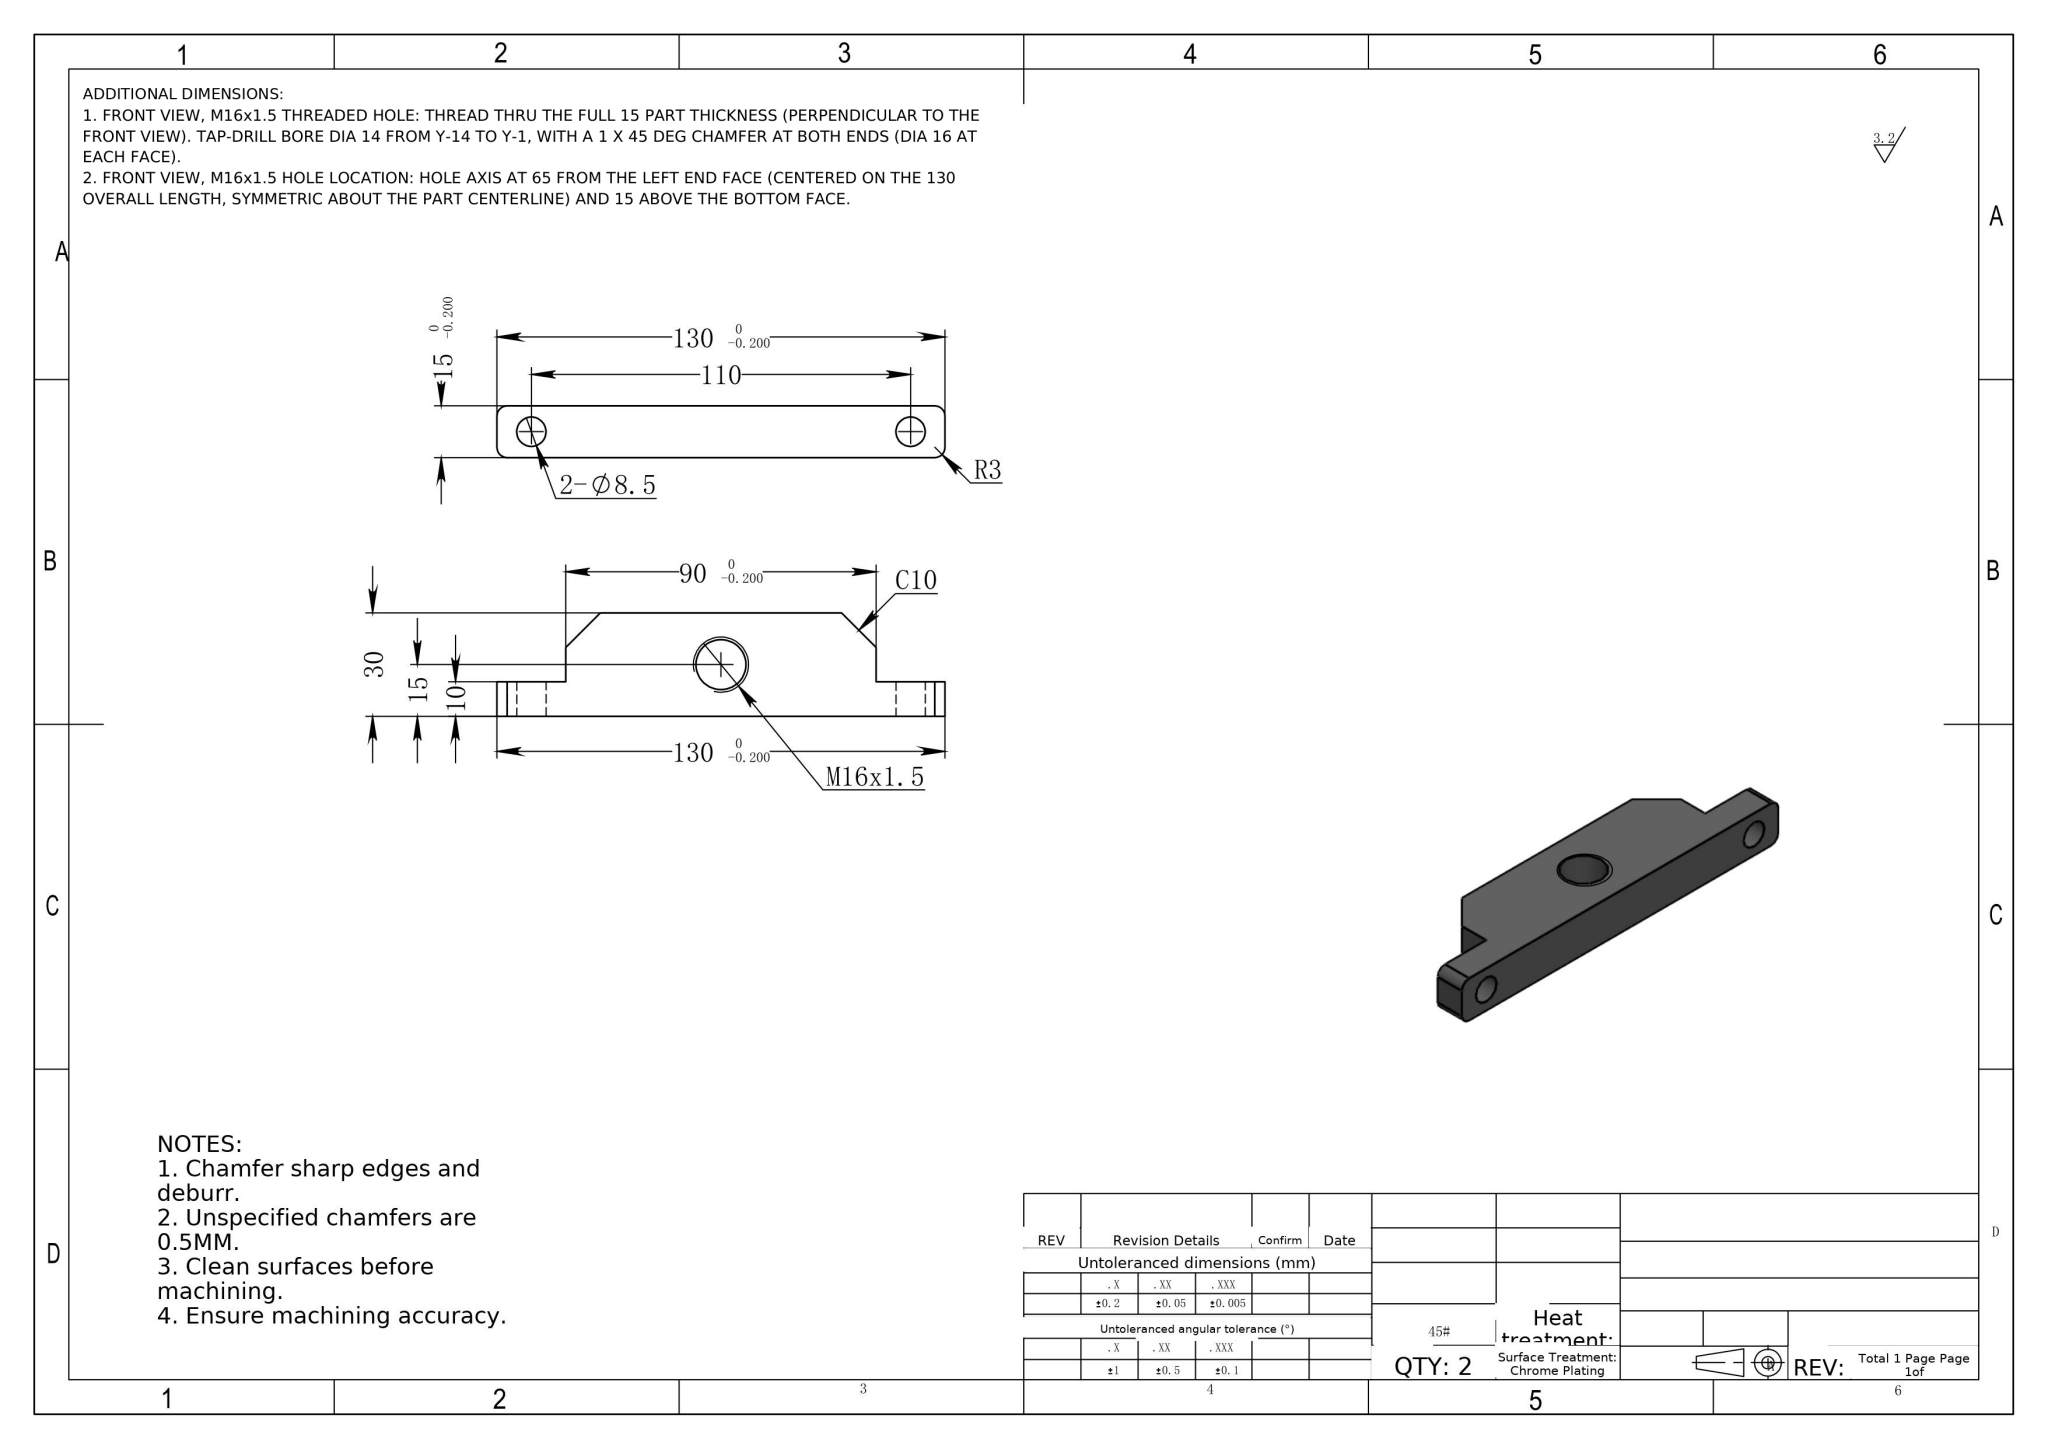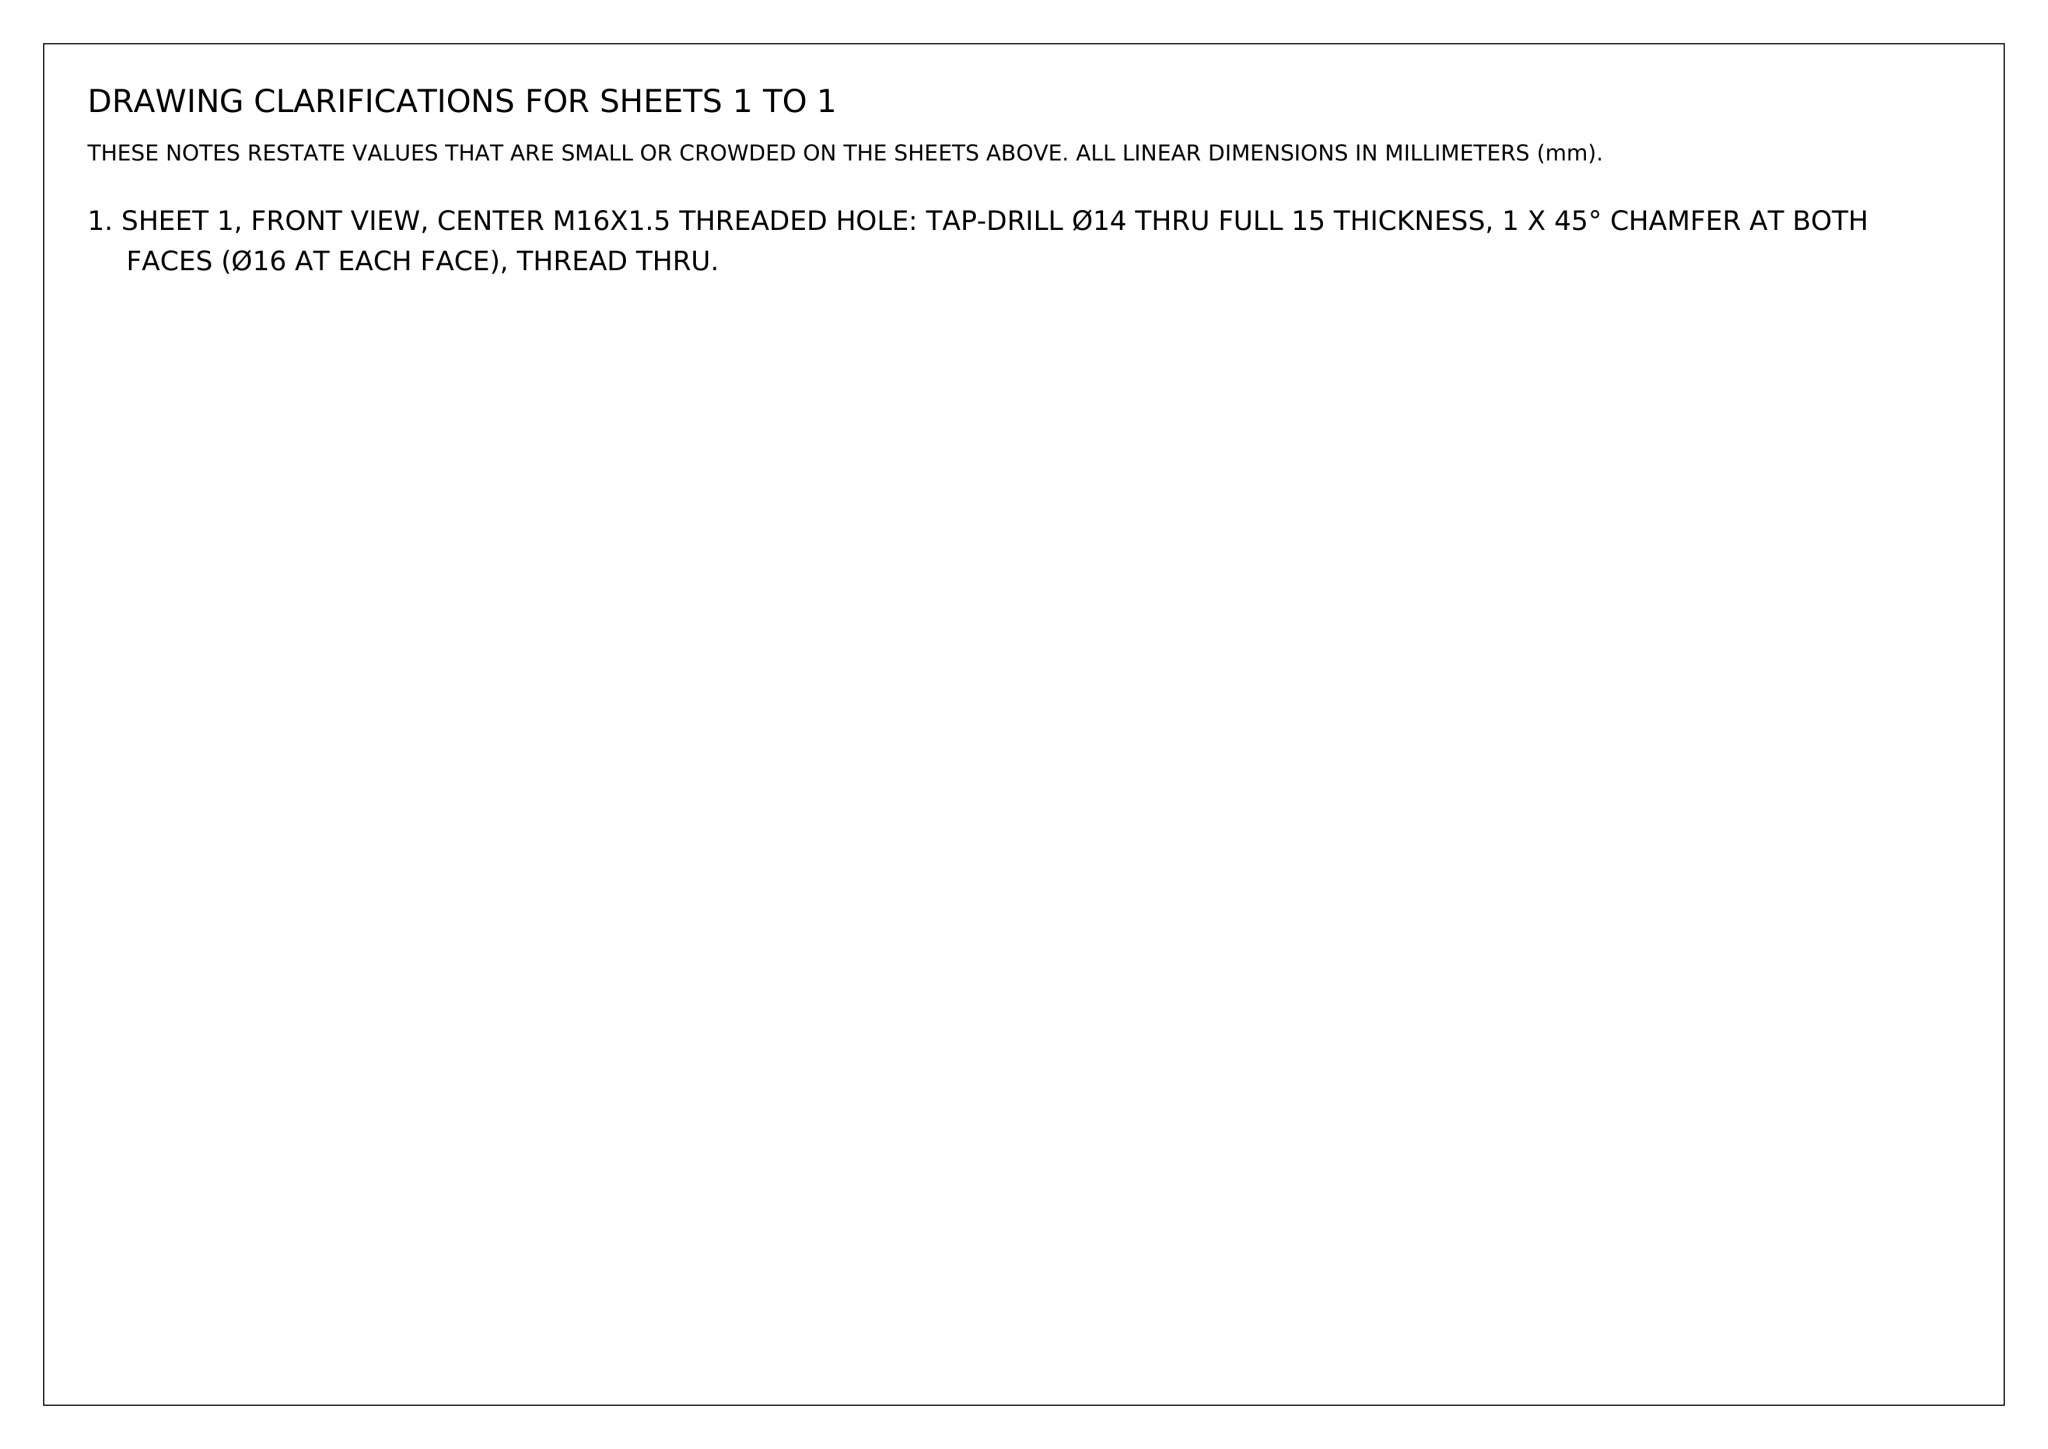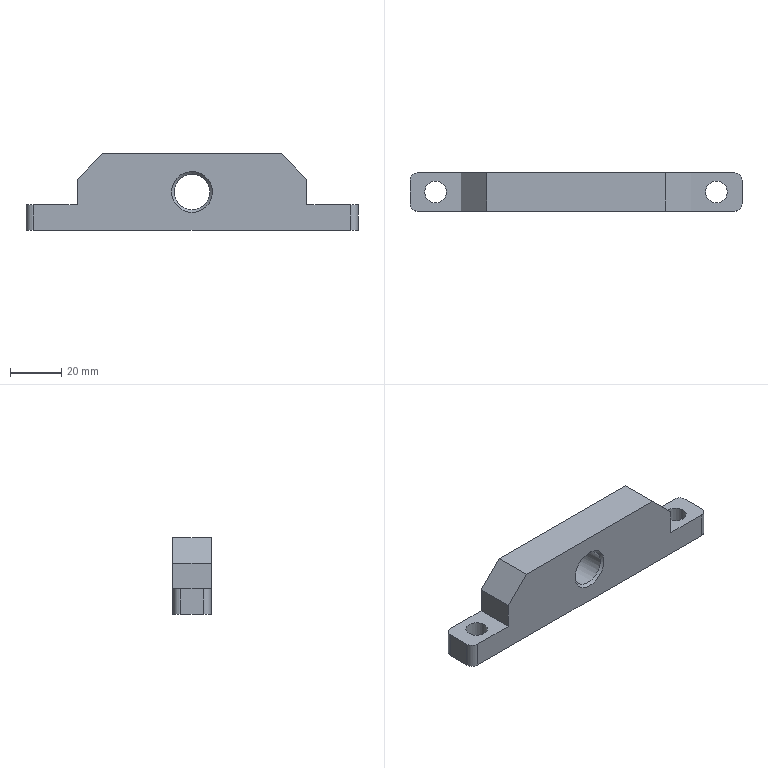Part | NX | mm | Offset Dual-Ear Mounting Bar | 1 solid | 21 faces | box 130 x 15 x 30 mm | volume 41433 mm3 | plane 12 | cylinder 7 | cone 2 | commonest cylinder face diameters 6 x4 8.5 x2 14 x1
STEP:
#1=CARTESIAN_POINT('',(0.,0.,0.));
#2=DIRECTION('',(0.,0.,1.));
#3=DIRECTION('',(1.,0.,0.));
#4=AXIS2_PLACEMENT_3D('',#1,#2,#3);
#5=(LENGTH_UNIT()NAMED_UNIT(*)SI_UNIT(.MILLI.,.METRE.));
#6=UNCERTAINTY_MEASURE_WITH_UNIT(LENGTH_MEASURE(0.00002),#5,'','');
#7=(NAMED_UNIT(*)PLANE_ANGLE_UNIT()SI_UNIT($,.RADIAN.));
#8=PLANE_ANGLE_MEASURE_WITH_UNIT(PLANE_ANGLE_MEASURE(0.01745),#7);
#9=DIMENSIONAL_EXPONENTS(0.,0.,0.,0.,0.,0.,0.);
#10=(CONVERSION_BASED_UNIT('',#8)NAMED_UNIT(#9)PLANE_ANGLE_UNIT());
#11=(NAMED_UNIT(*)SI_UNIT($,.STERADIAN.)SOLID_ANGLE_UNIT());
#12=(GEOMETRIC_REPRESENTATION_CONTEXT(3)GLOBAL_UNCERTAINTY_ASSIGNED_CONTEXT((#6))GLOBAL_UNIT_ASSIGNED_CONTEXT((#5,#10,#11))REPRESENTATION_CONTEXT('',''));
#13=SHAPE_REPRESENTATION('',(#4),#12);
#14=CARTESIAN_POINT('',(14.25,-7.5,10.));
#15=VERTEX_POINT('',#14);
#16=CARTESIAN_POINT('',(10.,-7.5,10.));
#17=DIRECTION('',(0.,0.,1.));
#18=DIRECTION('',(1.,0.,0.));
#19=AXIS2_PLACEMENT_3D('',#16,#17,#18);
#20=CIRCLE('',#19,4.25);
#21=EDGE_CURVE('',#15,#15,#20,.T.);
#22=ORIENTED_EDGE('',*,*,#21,.F.);
#23=EDGE_LOOP('',(#22));
#24=FACE_BOUND('',#23,.T.);
#25=CARTESIAN_POINT('',(20.,0.,10.));
#26=VERTEX_POINT('',#25);
#27=CARTESIAN_POINT('',(20.,-15.,10.));
#28=VERTEX_POINT('',#27);
#29=CARTESIAN_POINT('',(20.,0.,10.));
#30=DIRECTION('',(0.,-1.,0.));
#31=VECTOR('',#30,1.);
#32=LINE('',#29,#31);
#33=EDGE_CURVE('',#26,#28,#32,.T.);
#34=ORIENTED_EDGE('',*,*,#33,.F.);
#35=CARTESIAN_POINT('',(3.,0.,10.));
#36=VERTEX_POINT('',#35);
#37=CARTESIAN_POINT('',(130.,0.,10.));
#38=DIRECTION('',(-1.,-0.,0.));
#39=VECTOR('',#38,1.);
#40=LINE('',#37,#39);
#41=EDGE_CURVE('',#26,#36,#40,.T.);
#42=ORIENTED_EDGE('',*,*,#41,.T.);
#43=CARTESIAN_POINT('',(0.,-3.,10.));
#44=VERTEX_POINT('',#43);
#45=CARTESIAN_POINT('',(3.,-3.,10.));
#46=DIRECTION('',(0.,0.,1.));
#47=DIRECTION('',(1.,0.,0.));
#48=AXIS2_PLACEMENT_3D('',#45,#46,#47);
#49=CIRCLE('',#48,3.);
#50=EDGE_CURVE('',#36,#44,#49,.T.);
#51=ORIENTED_EDGE('',*,*,#50,.T.);
#52=CARTESIAN_POINT('',(0.,-12.,10.));
#53=VERTEX_POINT('',#52);
#54=CARTESIAN_POINT('',(0.,0.,10.));
#55=DIRECTION('',(0.,-1.,0.));
#56=VECTOR('',#55,1.);
#57=LINE('',#54,#56);
#58=EDGE_CURVE('',#44,#53,#57,.T.);
#59=ORIENTED_EDGE('',*,*,#58,.T.);
#60=CARTESIAN_POINT('',(3.,-15.,10.));
#61=VERTEX_POINT('',#60);
#62=CARTESIAN_POINT('',(3.,-12.,10.));
#63=DIRECTION('',(0.,0.,1.));
#64=DIRECTION('',(1.,0.,0.));
#65=AXIS2_PLACEMENT_3D('',#62,#63,#64);
#66=CIRCLE('',#65,3.);
#67=EDGE_CURVE('',#53,#61,#66,.T.);
#68=ORIENTED_EDGE('',*,*,#67,.T.);
#69=CARTESIAN_POINT('',(0.,-15.,10.));
#70=DIRECTION('',(1.,0.,0.));
#71=VECTOR('',#70,1.);
#72=LINE('',#69,#71);
#73=EDGE_CURVE('',#61,#28,#72,.T.);
#74=ORIENTED_EDGE('',*,*,#73,.T.);
#75=EDGE_LOOP('',(#34,#42,#51,#59,#68,#74));
#76=FACE_BOUND('',#75,.T.);
#77=CARTESIAN_POINT('',(0.,0.,10.));
#78=DIRECTION('',(0.,0.,1.));
#79=DIRECTION('',(1.,0.,0.));
#80=AXIS2_PLACEMENT_3D('',#77,#78,#79);
#81=PLANE('',#80);
#82=ADVANCED_FACE('',(#24,#76),#81,.T.);
#83=ORIENTED_EDGE('',*,*,#58,.F.);
#84=CARTESIAN_POINT('',(0.,-3.,0.));
#85=VERTEX_POINT('',#84);
#86=CARTESIAN_POINT('',(0.,-3.,10.));
#87=DIRECTION('',(0.,0.,-1.));
#88=VECTOR('',#87,1.);
#89=LINE('',#86,#88);
#90=EDGE_CURVE('',#44,#85,#89,.T.);
#91=ORIENTED_EDGE('',*,*,#90,.T.);
#92=CARTESIAN_POINT('',(0.,-12.,0.));
#93=VERTEX_POINT('',#92);
#94=CARTESIAN_POINT('',(0.,0.,0.));
#95=DIRECTION('',(0.,-1.,0.));
#96=VECTOR('',#95,1.);
#97=LINE('',#94,#96);
#98=EDGE_CURVE('',#85,#93,#97,.T.);
#99=ORIENTED_EDGE('',*,*,#98,.T.);
#100=CARTESIAN_POINT('',(0.,-12.,10.));
#101=DIRECTION('',(0.,0.,1.));
#102=VECTOR('',#101,1.);
#103=LINE('',#100,#102);
#104=EDGE_CURVE('',#93,#53,#103,.T.);
#105=ORIENTED_EDGE('',*,*,#104,.T.);
#106=EDGE_LOOP('',(#83,#91,#99,#105));
#107=FACE_OUTER_BOUND('',#106,.T.);
#108=CARTESIAN_POINT('',(0.,0.,10.));
#109=DIRECTION('',(1.,0.,0.));
#110=DIRECTION('',(0.,0.,-1.));
#111=AXIS2_PLACEMENT_3D('',#108,#109,#110);
#112=PLANE('',#111);
#113=ADVANCED_FACE('',(#107),#112,.F.);
#114=CARTESIAN_POINT('',(57.,-15.,15.));
#115=VERTEX_POINT('',#114);
#116=CARTESIAN_POINT('',(65.,-15.,15.));
#117=DIRECTION('',(-0.,1.,0.));
#118=DIRECTION('',(-1.,-0.,0.));
#119=AXIS2_PLACEMENT_3D('',#116,#117,#118);
#120=CIRCLE('',#119,8.);
#121=EDGE_CURVE('',#115,#115,#120,.T.);
#122=ORIENTED_EDGE('',*,*,#121,.T.);
#123=EDGE_LOOP('',(#122));
#124=FACE_BOUND('',#123,.T.);
#125=CARTESIAN_POINT('',(110.,-15.,20.));
#126=VERTEX_POINT('',#125);
#127=CARTESIAN_POINT('',(110.,-15.,10.));
#128=VERTEX_POINT('',#127);
#129=CARTESIAN_POINT('',(110.,-15.,30.));
#130=DIRECTION('',(0.,0.,-1.));
#131=VECTOR('',#130,1.);
#132=LINE('',#129,#131);
#133=EDGE_CURVE('',#126,#128,#132,.T.);
#134=ORIENTED_EDGE('',*,*,#133,.F.);
#135=CARTESIAN_POINT('',(100.,-15.,30.));
#136=VERTEX_POINT('',#135);
#137=CARTESIAN_POINT('',(100.,-15.,30.));
#138=DIRECTION('',(-0.7071,-0.,0.7071));
#139=VECTOR('',#138,1.);
#140=LINE('',#137,#139);
#141=EDGE_CURVE('',#126,#136,#140,.T.);
#142=ORIENTED_EDGE('',*,*,#141,.T.);
#143=CARTESIAN_POINT('',(30.,-15.,30.));
#144=VERTEX_POINT('',#143);
#145=CARTESIAN_POINT('',(20.,-15.,30.));
#146=DIRECTION('',(1.,0.,0.));
#147=VECTOR('',#146,1.);
#148=LINE('',#145,#147);
#149=EDGE_CURVE('',#144,#136,#148,.T.);
#150=ORIENTED_EDGE('',*,*,#149,.F.);
#151=CARTESIAN_POINT('',(20.,-15.,20.));
#152=VERTEX_POINT('',#151);
#153=CARTESIAN_POINT('',(30.,-15.,30.));
#154=DIRECTION('',(-0.7071,-0.,-0.7071));
#155=VECTOR('',#154,1.);
#156=LINE('',#153,#155);
#157=EDGE_CURVE('',#144,#152,#156,.T.);
#158=ORIENTED_EDGE('',*,*,#157,.T.);
#159=CARTESIAN_POINT('',(20.,-15.,30.));
#160=DIRECTION('',(0.,0.,-1.));
#161=VECTOR('',#160,1.);
#162=LINE('',#159,#161);
#163=EDGE_CURVE('',#152,#28,#162,.T.);
#164=ORIENTED_EDGE('',*,*,#163,.T.);
#165=ORIENTED_EDGE('',*,*,#73,.F.);
#166=CARTESIAN_POINT('',(3.,-15.,0.));
#167=VERTEX_POINT('',#166);
#168=CARTESIAN_POINT('',(3.,-15.,10.));
#169=DIRECTION('',(0.,0.,-1.));
#170=VECTOR('',#169,1.);
#171=LINE('',#168,#170);
#172=EDGE_CURVE('',#61,#167,#171,.T.);
#173=ORIENTED_EDGE('',*,*,#172,.T.);
#174=CARTESIAN_POINT('',(127.,-15.,0.));
#175=VERTEX_POINT('',#174);
#176=CARTESIAN_POINT('',(0.,-15.,0.));
#177=DIRECTION('',(1.,0.,0.));
#178=VECTOR('',#177,1.);
#179=LINE('',#176,#178);
#180=EDGE_CURVE('',#167,#175,#179,.T.);
#181=ORIENTED_EDGE('',*,*,#180,.T.);
#182=CARTESIAN_POINT('',(127.,-15.,10.));
#183=VERTEX_POINT('',#182);
#184=CARTESIAN_POINT('',(127.,-15.,10.));
#185=DIRECTION('',(0.,0.,1.));
#186=VECTOR('',#185,1.);
#187=LINE('',#184,#186);
#188=EDGE_CURVE('',#175,#183,#187,.T.);
#189=ORIENTED_EDGE('',*,*,#188,.T.);
#190=CARTESIAN_POINT('',(0.,-15.,10.));
#191=DIRECTION('',(1.,0.,0.));
#192=VECTOR('',#191,1.);
#193=LINE('',#190,#192);
#194=EDGE_CURVE('',#128,#183,#193,.T.);
#195=ORIENTED_EDGE('',*,*,#194,.F.);
#196=EDGE_LOOP('',(#134,#142,#150,#158,#164,#165,#173,#181,#189,#195));
#197=FACE_BOUND('',#196,.T.);
#198=CARTESIAN_POINT('',(0.,-15.,10.));
#199=DIRECTION('',(-0.,1.,0.));
#200=DIRECTION('',(-1.,-0.,0.));
#201=AXIS2_PLACEMENT_3D('',#198,#199,#200);
#202=PLANE('',#201);
#203=ADVANCED_FACE('',(#124,#197),#202,.F.);
#204=CARTESIAN_POINT('',(130.,-12.,0.));
#205=VERTEX_POINT('',#204);
#206=CARTESIAN_POINT('',(130.,-3.,0.));
#207=VERTEX_POINT('',#206);
#208=CARTESIAN_POINT('',(130.,-15.,0.));
#209=DIRECTION('',(0.,1.,0.));
#210=VECTOR('',#209,1.);
#211=LINE('',#208,#210);
#212=EDGE_CURVE('',#205,#207,#211,.T.);
#213=ORIENTED_EDGE('',*,*,#212,.T.);
#214=CARTESIAN_POINT('',(130.,-3.,10.));
#215=VERTEX_POINT('',#214);
#216=CARTESIAN_POINT('',(130.,-3.,10.));
#217=DIRECTION('',(0.,0.,1.));
#218=VECTOR('',#217,1.);
#219=LINE('',#216,#218);
#220=EDGE_CURVE('',#207,#215,#219,.T.);
#221=ORIENTED_EDGE('',*,*,#220,.T.);
#222=CARTESIAN_POINT('',(130.,-12.,10.));
#223=VERTEX_POINT('',#222);
#224=CARTESIAN_POINT('',(130.,-15.,10.));
#225=DIRECTION('',(0.,1.,0.));
#226=VECTOR('',#225,1.);
#227=LINE('',#224,#226);
#228=EDGE_CURVE('',#223,#215,#227,.T.);
#229=ORIENTED_EDGE('',*,*,#228,.F.);
#230=CARTESIAN_POINT('',(130.,-12.,10.));
#231=DIRECTION('',(0.,0.,-1.));
#232=VECTOR('',#231,1.);
#233=LINE('',#230,#232);
#234=EDGE_CURVE('',#223,#205,#233,.T.);
#235=ORIENTED_EDGE('',*,*,#234,.T.);
#236=EDGE_LOOP('',(#213,#221,#229,#235));
#237=FACE_OUTER_BOUND('',#236,.T.);
#238=CARTESIAN_POINT('',(130.,-15.,10.));
#239=DIRECTION('',(-1.,0.,0.));
#240=DIRECTION('',(0.,0.,1.));
#241=AXIS2_PLACEMENT_3D('',#238,#239,#240);
#242=PLANE('',#241);
#243=ADVANCED_FACE('',(#237),#242,.F.);
#244=CARTESIAN_POINT('',(73.,0.,15.));
#245=VERTEX_POINT('',#244);
#246=CARTESIAN_POINT('',(65.,0.,15.));
#247=DIRECTION('',(0.,-1.,0.));
#248=DIRECTION('',(1.,0.,0.));
#249=AXIS2_PLACEMENT_3D('',#246,#247,#248);
#250=CIRCLE('',#249,8.);
#251=EDGE_CURVE('',#245,#245,#250,.T.);
#252=ORIENTED_EDGE('',*,*,#251,.T.);
#253=EDGE_LOOP('',(#252));
#254=FACE_BOUND('',#253,.T.);
#255=CARTESIAN_POINT('',(100.,0.,30.));
#256=VERTEX_POINT('',#255);
#257=CARTESIAN_POINT('',(30.,0.,30.));
#258=VERTEX_POINT('',#257);
#259=CARTESIAN_POINT('',(110.,0.,30.));
#260=DIRECTION('',(-1.,-0.,0.));
#261=VECTOR('',#260,1.);
#262=LINE('',#259,#261);
#263=EDGE_CURVE('',#256,#258,#262,.T.);
#264=ORIENTED_EDGE('',*,*,#263,.F.);
#265=CARTESIAN_POINT('',(110.,0.,20.));
#266=VERTEX_POINT('',#265);
#267=CARTESIAN_POINT('',(100.,0.,30.));
#268=DIRECTION('',(0.7071,0.,-0.7071));
#269=VECTOR('',#268,1.);
#270=LINE('',#267,#269);
#271=EDGE_CURVE('',#256,#266,#270,.T.);
#272=ORIENTED_EDGE('',*,*,#271,.T.);
#273=CARTESIAN_POINT('',(110.,0.,10.));
#274=VERTEX_POINT('',#273);
#275=CARTESIAN_POINT('',(110.,0.,30.));
#276=DIRECTION('',(0.,0.,-1.));
#277=VECTOR('',#276,1.);
#278=LINE('',#275,#277);
#279=EDGE_CURVE('',#266,#274,#278,.T.);
#280=ORIENTED_EDGE('',*,*,#279,.T.);
#281=CARTESIAN_POINT('',(127.,0.,10.));
#282=VERTEX_POINT('',#281);
#283=CARTESIAN_POINT('',(130.,0.,10.));
#284=DIRECTION('',(-1.,-0.,0.));
#285=VECTOR('',#284,1.);
#286=LINE('',#283,#285);
#287=EDGE_CURVE('',#282,#274,#286,.T.);
#288=ORIENTED_EDGE('',*,*,#287,.F.);
#289=CARTESIAN_POINT('',(127.,0.,0.));
#290=VERTEX_POINT('',#289);
#291=CARTESIAN_POINT('',(127.,0.,10.));
#292=DIRECTION('',(0.,0.,-1.));
#293=VECTOR('',#292,1.);
#294=LINE('',#291,#293);
#295=EDGE_CURVE('',#282,#290,#294,.T.);
#296=ORIENTED_EDGE('',*,*,#295,.T.);
#297=CARTESIAN_POINT('',(3.,0.,0.));
#298=VERTEX_POINT('',#297);
#299=CARTESIAN_POINT('',(130.,0.,0.));
#300=DIRECTION('',(-1.,-0.,0.));
#301=VECTOR('',#300,1.);
#302=LINE('',#299,#301);
#303=EDGE_CURVE('',#290,#298,#302,.T.);
#304=ORIENTED_EDGE('',*,*,#303,.T.);
#305=CARTESIAN_POINT('',(3.,0.,10.));
#306=DIRECTION('',(0.,0.,1.));
#307=VECTOR('',#306,1.);
#308=LINE('',#305,#307);
#309=EDGE_CURVE('',#298,#36,#308,.T.);
#310=ORIENTED_EDGE('',*,*,#309,.T.);
#311=ORIENTED_EDGE('',*,*,#41,.F.);
#312=CARTESIAN_POINT('',(20.,0.,20.));
#313=VERTEX_POINT('',#312);
#314=CARTESIAN_POINT('',(20.,0.,30.));
#315=DIRECTION('',(0.,0.,-1.));
#316=VECTOR('',#315,1.);
#317=LINE('',#314,#316);
#318=EDGE_CURVE('',#313,#26,#317,.T.);
#319=ORIENTED_EDGE('',*,*,#318,.F.);
#320=CARTESIAN_POINT('',(30.,0.,30.));
#321=DIRECTION('',(0.7071,0.,0.7071));
#322=VECTOR('',#321,1.);
#323=LINE('',#320,#322);
#324=EDGE_CURVE('',#313,#258,#323,.T.);
#325=ORIENTED_EDGE('',*,*,#324,.T.);
#326=EDGE_LOOP('',(#264,#272,#280,#288,#296,#304,#310,#311,#319,#325));
#327=FACE_BOUND('',#326,.T.);
#328=CARTESIAN_POINT('',(130.,0.,10.));
#329=DIRECTION('',(0.,-1.,0.));
#330=DIRECTION('',(1.,0.,0.));
#331=AXIS2_PLACEMENT_3D('',#328,#329,#330);
#332=PLANE('',#331);
#333=ADVANCED_FACE('',(#254,#327),#332,.F.);
#334=CARTESIAN_POINT('',(124.25,-7.5,10.));
#335=VERTEX_POINT('',#334);
#336=CARTESIAN_POINT('',(120.,-7.5,10.));
#337=DIRECTION('',(0.,0.,1.));
#338=DIRECTION('',(1.,0.,0.));
#339=AXIS2_PLACEMENT_3D('',#336,#337,#338);
#340=CIRCLE('',#339,4.25);
#341=EDGE_CURVE('',#335,#335,#340,.T.);
#342=ORIENTED_EDGE('',*,*,#341,.F.);
#343=EDGE_LOOP('',(#342));
#344=FACE_BOUND('',#343,.T.);
#345=CARTESIAN_POINT('',(110.,-15.,10.));
#346=DIRECTION('',(0.,1.,0.));
#347=VECTOR('',#346,1.);
#348=LINE('',#345,#347);
#349=EDGE_CURVE('',#128,#274,#348,.T.);
#350=ORIENTED_EDGE('',*,*,#349,.F.);
#351=ORIENTED_EDGE('',*,*,#194,.T.);
#352=CARTESIAN_POINT('',(127.,-12.,10.));
#353=DIRECTION('',(0.,0.,1.));
#354=DIRECTION('',(1.,0.,0.));
#355=AXIS2_PLACEMENT_3D('',#352,#353,#354);
#356=CIRCLE('',#355,3.);
#357=EDGE_CURVE('',#183,#223,#356,.T.);
#358=ORIENTED_EDGE('',*,*,#357,.T.);
#359=ORIENTED_EDGE('',*,*,#228,.T.);
#360=CARTESIAN_POINT('',(127.,-3.,10.));
#361=DIRECTION('',(0.,0.,1.));
#362=DIRECTION('',(1.,0.,0.));
#363=AXIS2_PLACEMENT_3D('',#360,#361,#362);
#364=CIRCLE('',#363,3.);
#365=EDGE_CURVE('',#215,#282,#364,.T.);
#366=ORIENTED_EDGE('',*,*,#365,.T.);
#367=ORIENTED_EDGE('',*,*,#287,.T.);
#368=EDGE_LOOP('',(#350,#351,#358,#359,#366,#367));
#369=FACE_BOUND('',#368,.T.);
#370=CARTESIAN_POINT('',(0.,0.,10.));
#371=DIRECTION('',(0.,0.,1.));
#372=DIRECTION('',(1.,0.,0.));
#373=AXIS2_PLACEMENT_3D('',#370,#371,#372);
#374=PLANE('',#373);
#375=ADVANCED_FACE('',(#344,#369),#374,.T.);
#376=CARTESIAN_POINT('',(124.25,-7.5,0.));
#377=VERTEX_POINT('',#376);
#378=CARTESIAN_POINT('',(120.,-7.5,0.));
#379=DIRECTION('',(0.,0.,-1.));
#380=DIRECTION('',(1.,0.,0.));
#381=AXIS2_PLACEMENT_3D('',#378,#379,#380);
#382=CIRCLE('',#381,4.25);
#383=EDGE_CURVE('',#377,#377,#382,.T.);
#384=ORIENTED_EDGE('',*,*,#383,.F.);
#385=EDGE_LOOP('',(#384));
#386=FACE_BOUND('',#385,.T.);
#387=CARTESIAN_POINT('',(14.25,-7.5,0.));
#388=VERTEX_POINT('',#387);
#389=CARTESIAN_POINT('',(10.,-7.5,0.));
#390=DIRECTION('',(0.,0.,-1.));
#391=DIRECTION('',(1.,0.,0.));
#392=AXIS2_PLACEMENT_3D('',#389,#390,#391);
#393=CIRCLE('',#392,4.25);
#394=EDGE_CURVE('',#388,#388,#393,.T.);
#395=ORIENTED_EDGE('',*,*,#394,.F.);
#396=EDGE_LOOP('',(#395));
#397=FACE_BOUND('',#396,.T.);
#398=ORIENTED_EDGE('',*,*,#98,.F.);
#399=CARTESIAN_POINT('',(3.,-3.,0.));
#400=DIRECTION('',(0.,0.,-1.));
#401=DIRECTION('',(1.,0.,0.));
#402=AXIS2_PLACEMENT_3D('',#399,#400,#401);
#403=CIRCLE('',#402,3.);
#404=EDGE_CURVE('',#85,#298,#403,.T.);
#405=ORIENTED_EDGE('',*,*,#404,.T.);
#406=ORIENTED_EDGE('',*,*,#303,.F.);
#407=CARTESIAN_POINT('',(127.,-3.,0.));
#408=DIRECTION('',(0.,0.,-1.));
#409=DIRECTION('',(1.,0.,0.));
#410=AXIS2_PLACEMENT_3D('',#407,#408,#409);
#411=CIRCLE('',#410,3.);
#412=EDGE_CURVE('',#290,#207,#411,.T.);
#413=ORIENTED_EDGE('',*,*,#412,.T.);
#414=ORIENTED_EDGE('',*,*,#212,.F.);
#415=CARTESIAN_POINT('',(127.,-12.,0.));
#416=DIRECTION('',(0.,0.,-1.));
#417=DIRECTION('',(1.,0.,0.));
#418=AXIS2_PLACEMENT_3D('',#415,#416,#417);
#419=CIRCLE('',#418,3.);
#420=EDGE_CURVE('',#205,#175,#419,.T.);
#421=ORIENTED_EDGE('',*,*,#420,.T.);
#422=ORIENTED_EDGE('',*,*,#180,.F.);
#423=CARTESIAN_POINT('',(3.,-12.,0.));
#424=DIRECTION('',(0.,0.,-1.));
#425=DIRECTION('',(1.,0.,0.));
#426=AXIS2_PLACEMENT_3D('',#423,#424,#425);
#427=CIRCLE('',#426,3.);
#428=EDGE_CURVE('',#167,#93,#427,.T.);
#429=ORIENTED_EDGE('',*,*,#428,.T.);
#430=EDGE_LOOP('',(#398,#405,#406,#413,#414,#421,#422,#429));
#431=FACE_BOUND('',#430,.T.);
#432=CARTESIAN_POINT('',(0.,0.,0.));
#433=DIRECTION('',(0.,0.,1.));
#434=DIRECTION('',(1.,0.,0.));
#435=AXIS2_PLACEMENT_3D('',#432,#433,#434);
#436=PLANE('',#435);
#437=ADVANCED_FACE('',(#386,#397,#431),#436,.F.);
#438=ORIENTED_EDGE('',*,*,#50,.F.);
#439=ORIENTED_EDGE('',*,*,#309,.F.);
#440=ORIENTED_EDGE('',*,*,#404,.F.);
#441=ORIENTED_EDGE('',*,*,#90,.F.);
#442=EDGE_LOOP('',(#438,#439,#440,#441));
#443=FACE_OUTER_BOUND('',#442,.T.);
#444=CARTESIAN_POINT('',(3.,-3.,10.));
#445=DIRECTION('',(0.,0.,-1.));
#446=DIRECTION('',(-1.,0.,0.));
#447=AXIS2_PLACEMENT_3D('',#444,#445,#446);
#448=CYLINDRICAL_SURFACE('',#447,3.);
#449=ADVANCED_FACE('',(#443),#448,.T.);
#450=ORIENTED_EDGE('',*,*,#67,.F.);
#451=ORIENTED_EDGE('',*,*,#104,.F.);
#452=ORIENTED_EDGE('',*,*,#428,.F.);
#453=ORIENTED_EDGE('',*,*,#172,.F.);
#454=EDGE_LOOP('',(#450,#451,#452,#453));
#455=FACE_OUTER_BOUND('',#454,.T.);
#456=CARTESIAN_POINT('',(3.,-12.,10.));
#457=DIRECTION('',(0.,0.,-1.));
#458=DIRECTION('',(-1.,0.,0.));
#459=AXIS2_PLACEMENT_3D('',#456,#457,#458);
#460=CYLINDRICAL_SURFACE('',#459,3.);
#461=ADVANCED_FACE('',(#455),#460,.T.);
#462=ORIENTED_EDGE('',*,*,#365,.F.);
#463=ORIENTED_EDGE('',*,*,#220,.F.);
#464=ORIENTED_EDGE('',*,*,#412,.F.);
#465=ORIENTED_EDGE('',*,*,#295,.F.);
#466=EDGE_LOOP('',(#462,#463,#464,#465));
#467=FACE_OUTER_BOUND('',#466,.T.);
#468=CARTESIAN_POINT('',(127.,-3.,10.));
#469=DIRECTION('',(0.,0.,-1.));
#470=DIRECTION('',(-1.,0.,0.));
#471=AXIS2_PLACEMENT_3D('',#468,#469,#470);
#472=CYLINDRICAL_SURFACE('',#471,3.);
#473=ADVANCED_FACE('',(#467),#472,.T.);
#474=ORIENTED_EDGE('',*,*,#357,.F.);
#475=ORIENTED_EDGE('',*,*,#188,.F.);
#476=ORIENTED_EDGE('',*,*,#420,.F.);
#477=ORIENTED_EDGE('',*,*,#234,.F.);
#478=EDGE_LOOP('',(#474,#475,#476,#477));
#479=FACE_OUTER_BOUND('',#478,.T.);
#480=CARTESIAN_POINT('',(127.,-12.,10.));
#481=DIRECTION('',(0.,0.,-1.));
#482=DIRECTION('',(-1.,0.,0.));
#483=AXIS2_PLACEMENT_3D('',#480,#481,#482);
#484=CYLINDRICAL_SURFACE('',#483,3.);
#485=ADVANCED_FACE('',(#479),#484,.T.);
#486=ORIENTED_EDGE('',*,*,#163,.F.);
#487=CARTESIAN_POINT('',(20.,0.,20.));
#488=DIRECTION('',(0.,1.,0.));
#489=VECTOR('',#488,1.);
#490=LINE('',#487,#489);
#491=EDGE_CURVE('',#152,#313,#490,.T.);
#492=ORIENTED_EDGE('',*,*,#491,.T.);
#493=ORIENTED_EDGE('',*,*,#318,.T.);
#494=ORIENTED_EDGE('',*,*,#33,.T.);
#495=EDGE_LOOP('',(#486,#492,#493,#494));
#496=FACE_OUTER_BOUND('',#495,.T.);
#497=CARTESIAN_POINT('',(20.,0.,30.));
#498=DIRECTION('',(1.,0.,0.));
#499=DIRECTION('',(0.,0.,-1.));
#500=AXIS2_PLACEMENT_3D('',#497,#498,#499);
#501=PLANE('',#500);
#502=ADVANCED_FACE('',(#496),#501,.F.);
#503=ORIENTED_EDGE('',*,*,#279,.F.);
#504=CARTESIAN_POINT('',(110.,-15.,20.));
#505=DIRECTION('',(-0.,-1.,0.));
#506=VECTOR('',#505,1.);
#507=LINE('',#504,#506);
#508=EDGE_CURVE('',#266,#126,#507,.T.);
#509=ORIENTED_EDGE('',*,*,#508,.T.);
#510=ORIENTED_EDGE('',*,*,#133,.T.);
#511=ORIENTED_EDGE('',*,*,#349,.T.);
#512=EDGE_LOOP('',(#503,#509,#510,#511));
#513=FACE_OUTER_BOUND('',#512,.T.);
#514=CARTESIAN_POINT('',(110.,-15.,30.));
#515=DIRECTION('',(-1.,0.,0.));
#516=DIRECTION('',(-0.,-1.,0.));
#517=AXIS2_PLACEMENT_3D('',#514,#515,#516);
#518=PLANE('',#517);
#519=ADVANCED_FACE('',(#513),#518,.F.);
#520=ORIENTED_EDGE('',*,*,#149,.T.);
#521=CARTESIAN_POINT('',(100.,0.,30.));
#522=DIRECTION('',(0.,1.,0.));
#523=VECTOR('',#522,1.);
#524=LINE('',#521,#523);
#525=EDGE_CURVE('',#136,#256,#524,.T.);
#526=ORIENTED_EDGE('',*,*,#525,.T.);
#527=ORIENTED_EDGE('',*,*,#263,.T.);
#528=CARTESIAN_POINT('',(30.,-15.,30.));
#529=DIRECTION('',(0.,-1.,0.));
#530=VECTOR('',#529,1.);
#531=LINE('',#528,#530);
#532=EDGE_CURVE('',#258,#144,#531,.T.);
#533=ORIENTED_EDGE('',*,*,#532,.T.);
#534=EDGE_LOOP('',(#520,#526,#527,#533));
#535=FACE_OUTER_BOUND('',#534,.T.);
#536=CARTESIAN_POINT('',(0.,0.,30.));
#537=DIRECTION('',(0.,0.,1.));
#538=DIRECTION('',(1.,0.,0.));
#539=AXIS2_PLACEMENT_3D('',#536,#537,#538);
#540=PLANE('',#539);
#541=ADVANCED_FACE('',(#535),#540,.T.);
#542=ORIENTED_EDGE('',*,*,#141,.F.);
#543=ORIENTED_EDGE('',*,*,#508,.F.);
#544=ORIENTED_EDGE('',*,*,#271,.F.);
#545=ORIENTED_EDGE('',*,*,#525,.F.);
#546=EDGE_LOOP('',(#542,#543,#544,#545));
#547=FACE_OUTER_BOUND('',#546,.T.);
#548=CARTESIAN_POINT('',(100.,-0.,30.));
#549=DIRECTION('',(0.7071,-0.,0.7071));
#550=DIRECTION('',(-0.,-1.,0.));
#551=AXIS2_PLACEMENT_3D('',#548,#549,#550);
#552=PLANE('',#551);
#553=ADVANCED_FACE('',(#547),#552,.T.);
#554=ORIENTED_EDGE('',*,*,#324,.F.);
#555=ORIENTED_EDGE('',*,*,#491,.F.);
#556=ORIENTED_EDGE('',*,*,#157,.F.);
#557=ORIENTED_EDGE('',*,*,#532,.F.);
#558=EDGE_LOOP('',(#554,#555,#556,#557));
#559=FACE_OUTER_BOUND('',#558,.T.);
#560=CARTESIAN_POINT('',(30.,0.,30.));
#561=DIRECTION('',(-0.7071,0.,0.7071));
#562=DIRECTION('',(0.,1.,0.));
#563=AXIS2_PLACEMENT_3D('',#560,#561,#562);
#564=PLANE('',#563);
#565=ADVANCED_FACE('',(#559),#564,.T.);
#566=ORIENTED_EDGE('',*,*,#21,.T.);
#567=EDGE_LOOP('',(#566));
#568=FACE_BOUND('',#567,.T.);
#569=ORIENTED_EDGE('',*,*,#394,.T.);
#570=EDGE_LOOP('',(#569));
#571=FACE_BOUND('',#570,.T.);
#572=CARTESIAN_POINT('',(10.,-7.5,20.));
#573=DIRECTION('',(0.,0.,-1.));
#574=DIRECTION('',(-1.,0.,0.));
#575=AXIS2_PLACEMENT_3D('',#572,#573,#574);
#576=CYLINDRICAL_SURFACE('',#575,4.25);
#577=ADVANCED_FACE('',(#568,#571),#576,.F.);
#578=ORIENTED_EDGE('',*,*,#341,.T.);
#579=EDGE_LOOP('',(#578));
#580=FACE_BOUND('',#579,.T.);
#581=ORIENTED_EDGE('',*,*,#383,.T.);
#582=EDGE_LOOP('',(#581));
#583=FACE_BOUND('',#582,.T.);
#584=CARTESIAN_POINT('',(120.,-7.5,20.));
#585=DIRECTION('',(0.,0.,-1.));
#586=DIRECTION('',(-1.,0.,0.));
#587=AXIS2_PLACEMENT_3D('',#584,#585,#586);
#588=CYLINDRICAL_SURFACE('',#587,4.25);
#589=ADVANCED_FACE('',(#580,#583),#588,.F.);
#590=CARTESIAN_POINT('',(65.,-1.,8.));
#591=VERTEX_POINT('',#590);
#592=CARTESIAN_POINT('',(65.,-1.,15.));
#593=DIRECTION('',(0.,1.,0.));
#594=DIRECTION('',(0.,0.,-1.));
#595=AXIS2_PLACEMENT_3D('',#592,#593,#594);
#596=CIRCLE('',#595,7.);
#597=EDGE_CURVE('',#591,#591,#596,.T.);
#598=ORIENTED_EDGE('',*,*,#597,.T.);
#599=EDGE_LOOP('',(#598));
#600=FACE_BOUND('',#599,.T.);
#601=CARTESIAN_POINT('',(65.,-14.,22.));
#602=VERTEX_POINT('',#601);
#603=CARTESIAN_POINT('',(65.,-14.,15.));
#604=DIRECTION('',(0.,-1.,0.));
#605=DIRECTION('',(0.,0.,1.));
#606=AXIS2_PLACEMENT_3D('',#603,#604,#605);
#607=CIRCLE('',#606,7.);
#608=EDGE_CURVE('',#602,#602,#607,.T.);
#609=ORIENTED_EDGE('',*,*,#608,.T.);
#610=EDGE_LOOP('',(#609));
#611=FACE_BOUND('',#610,.T.);
#612=CARTESIAN_POINT('',(65.,-15.,15.));
#613=DIRECTION('',(-0.,1.,0.));
#614=DIRECTION('',(-1.,-0.,0.));
#615=AXIS2_PLACEMENT_3D('',#612,#613,#614);
#616=CYLINDRICAL_SURFACE('',#615,7.);
#617=ADVANCED_FACE('',(#600,#611),#616,.F.);
#618=ORIENTED_EDGE('',*,*,#608,.F.);
#619=EDGE_LOOP('',(#618));
#620=FACE_BOUND('',#619,.T.);
#621=ORIENTED_EDGE('',*,*,#121,.F.);
#622=EDGE_LOOP('',(#621));
#623=FACE_BOUND('',#622,.T.);
#624=CARTESIAN_POINT('',(65.,-15.,15.));
#625=DIRECTION('',(0.,-1.,0.));
#626=DIRECTION('',(0.,0.,-1.));
#627=AXIS2_PLACEMENT_3D('',#624,#625,#626);
#628=CONICAL_SURFACE('',#627,8.,45.);
#629=ADVANCED_FACE('',(#620,#623),#628,.F.);
#630=ORIENTED_EDGE('',*,*,#251,.F.);
#631=EDGE_LOOP('',(#630));
#632=FACE_BOUND('',#631,.T.);
#633=ORIENTED_EDGE('',*,*,#597,.F.);
#634=EDGE_LOOP('',(#633));
#635=FACE_BOUND('',#634,.T.);
#636=CARTESIAN_POINT('',(65.,-1.,15.));
#637=DIRECTION('',(0.,1.,0.));
#638=DIRECTION('',(0.,-0.,1.));
#639=AXIS2_PLACEMENT_3D('',#636,#637,#638);
#640=CONICAL_SURFACE('',#639,7.,45.);
#641=ADVANCED_FACE('',(#632,#635),#640,.F.);
#642=CLOSED_SHELL('',(#82,#113,#203,#243,#333,#375,#437,#449,#461,#473,#485,#502,#519,#541,#553,#565,#577,#589,#617,#629,#641));
#643=MANIFOLD_SOLID_BREP('',#642);
#644=ADVANCED_BREP_SHAPE_REPRESENTATION('',(#643),#12);
#645=SHAPE_REPRESENTATION_RELATIONSHIP('','',#13,#644);
#646=PRESENTATION_LAYER_ASSIGNMENT('','',(#643));
#647=COLOUR_RGB('',1.,0.6,0.);
#648=FILL_AREA_STYLE_COLOUR('',#647);
#649=FILL_AREA_STYLE('',(#648));
#650=SURFACE_STYLE_FILL_AREA(#649);
#651=SURFACE_SIDE_STYLE('',(#650));
#652=SURFACE_STYLE_USAGE(.BOTH.,#651);
#653=PRESENTATION_STYLE_ASSIGNMENT((#652));
#654=STYLED_ITEM('',(#653),#643);
#655=MECHANICAL_DESIGN_GEOMETRIC_PRESENTATION_REPRESENTATION('',(#654),#12);